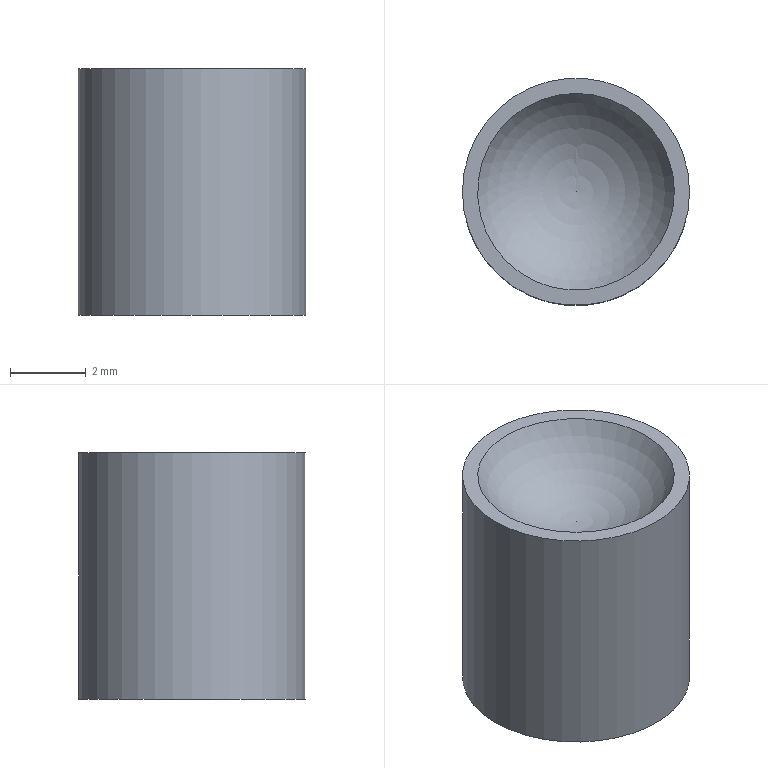Component | NX | DXF_02_SPRING_BRACKET | 1 solid | 4 faces | box 6 x 6 x 6.5 mm | volume 166 mm3 | plane 2 | cylinder 1 | sphere 1 | commonest cylinder face diameters 6 x1
STEP:
#1=CARTESIAN_POINT('',(0.,0.,0.));
#2=DIRECTION('',(0.,0.,1.));
#3=DIRECTION('',(1.,0.,0.));
#4=AXIS2_PLACEMENT_3D('',#1,#2,#3);
#5=CARTESIAN_POINT('',(3.,-0.,27.531));
#6=VERTEX_POINT('',#5);
#7=CARTESIAN_POINT('',(0.,-0.,27.531));
#8=DIRECTION('',(0.,0.,-1.));
#9=DIRECTION('',(1.,0.,0.));
#10=AXIS2_PLACEMENT_3D('',#7,#8,#9);
#11=CIRCLE('',#10,3.);
#12=CARTESIAN_POINT('',(0.,-0.,17.531));
#13=DIRECTION('',(0.,0.,1.));
#14=DIRECTION('',(1.,0.,0.));
#15=AXIS2_PLACEMENT_3D('',#12,#13,#14);
#16=CYLINDRICAL_SURFACE('',#15,3.);
#17=CARTESIAN_POINT('',(6.283,10.));
#18=DIRECTION('',(-1.,0.));
#19=VECTOR('',#18,1.);
#20=LINE('',#17,#19);
#21=(GEOMETRIC_REPRESENTATION_CONTEXT(2)PARAMETRIC_REPRESENTATION_CONTEXT()REPRESENTATION_CONTEXT('',''));
#22=DEFINITIONAL_REPRESENTATION('',(#20),#21);
#23=PCURVE('',#16,#22);
#24=CARTESIAN_POINT('',(0.,-0.,27.531));
#25=DIRECTION('',(0.,0.,1.));
#26=DIRECTION('',(1.,0.,0.));
#27=AXIS2_PLACEMENT_3D('',#24,#25,#26);
#28=PLANE('',#27);
#29=CARTESIAN_POINT('',(3.,0.));
#30=CARTESIAN_POINT('',(3.,-5.196));
#31=CARTESIAN_POINT('',(-1.5,-2.598));
#32=CARTESIAN_POINT('',(-6.,-0.));
#33=CARTESIAN_POINT('',(-1.5,2.598));
#34=CARTESIAN_POINT('',(3.,5.196));
#35=CARTESIAN_POINT('',(3.,0.));
#36=(BOUNDED_CURVE()B_SPLINE_CURVE(2,(#29,#30,#31,#32,#33,#34,#35),.UNSPECIFIED.,.T.,.F.)B_SPLINE_CURVE_WITH_KNOTS((1,2,2,2,2,1),(-2.094,0.,2.094,4.189,6.283,8.378),.UNSPECIFIED.)CURVE()GEOMETRIC_REPRESENTATION_ITEM()RATIONAL_B_SPLINE_CURVE((1.,0.5,1.,0.5,1.,0.5,1.))REPRESENTATION_ITEM(''));
#37=(GEOMETRIC_REPRESENTATION_CONTEXT(2)PARAMETRIC_REPRESENTATION_CONTEXT()REPRESENTATION_CONTEXT('',''));
#38=DEFINITIONAL_REPRESENTATION('',(#36),#37);
#39=PCURVE('',#28,#38);
#40=SURFACE_CURVE('',#11,(#23,#39),.PCURVE_S1.);
#41=EDGE_CURVE('',#6,#6,#40,.T.);
#42=ORIENTED_EDGE('',*,*,#41,.T.);
#43=CARTESIAN_POINT('',(3.,-0.,21.031));
#44=VERTEX_POINT('',#43);
#45=CARTESIAN_POINT('',(3.,-0.,21.031));
#46=CARTESIAN_POINT('',(3.,-0.,27.531));
#47=B_SPLINE_CURVE_WITH_KNOTS('',1,(#45,#46),.UNSPECIFIED.,.F.,.F.,(2,2),(3.5,10.),.PIECEWISE_BEZIER_KNOTS.);
#48=CARTESIAN_POINT('',(0.,0.));
#49=DIRECTION('',(0.,1.));
#50=VECTOR('',#49,1.);
#51=LINE('',#48,#50);
#52=(GEOMETRIC_REPRESENTATION_CONTEXT(2)PARAMETRIC_REPRESENTATION_CONTEXT()REPRESENTATION_CONTEXT('',''));
#53=DEFINITIONAL_REPRESENTATION('',(#51),#52);
#54=PCURVE('',#16,#53);
#55=CARTESIAN_POINT('',(6.283,0.));
#56=DIRECTION('',(0.,1.));
#57=VECTOR('',#56,1.);
#58=LINE('',#55,#57);
#59=(GEOMETRIC_REPRESENTATION_CONTEXT(2)PARAMETRIC_REPRESENTATION_CONTEXT()REPRESENTATION_CONTEXT('',''));
#60=DEFINITIONAL_REPRESENTATION('',(#58),#59);
#61=PCURVE('',#16,#60);
#62=SEAM_CURVE('',#47,(#54,#61),.PCURVE_S1.);
#63=EDGE_CURVE('',#44,#6,#62,.T.);
#64=ORIENTED_EDGE('',*,*,#63,.F.);
#65=CARTESIAN_POINT('',(-3.,-0.,21.031));
#66=VERTEX_POINT('',#65);
#67=CARTESIAN_POINT('',(0.,-0.,21.031));
#68=DIRECTION('',(0.,0.,1.));
#69=DIRECTION('',(-1.,0.,0.));
#70=AXIS2_PLACEMENT_3D('',#67,#68,#69);
#71=CIRCLE('',#70,3.);
#72=CARTESIAN_POINT('',(-3.142,3.5));
#73=DIRECTION('',(1.,0.));
#74=VECTOR('',#73,1.);
#75=LINE('',#72,#74);
#76=(GEOMETRIC_REPRESENTATION_CONTEXT(2)PARAMETRIC_REPRESENTATION_CONTEXT()REPRESENTATION_CONTEXT('',''));
#77=DEFINITIONAL_REPRESENTATION('',(#75),#76);
#78=PCURVE('',#16,#77);
#79=CARTESIAN_POINT('',(0.,-0.,21.031));
#80=DIRECTION('',(0.,0.,-1.));
#81=DIRECTION('',(-1.,0.,0.));
#82=AXIS2_PLACEMENT_3D('',#79,#80,#81);
#83=PLANE('',#82);
#84=CARTESIAN_POINT('',(3.,0.));
#85=CARTESIAN_POINT('',(3.,-5.196));
#86=CARTESIAN_POINT('',(-1.5,-2.598));
#87=CARTESIAN_POINT('',(-6.,-0.));
#88=CARTESIAN_POINT('',(-1.5,2.598));
#89=CARTESIAN_POINT('',(3.,5.196));
#90=CARTESIAN_POINT('',(3.,0.));
#91=(BOUNDED_CURVE()B_SPLINE_CURVE(2,(#84,#85,#86,#87,#88,#89,#90),.UNSPECIFIED.,.T.,.F.)B_SPLINE_CURVE_WITH_KNOTS((1,2,2,2,2,1),(-2.094,0.,2.094,4.189,6.283,8.378),.UNSPECIFIED.)CURVE()GEOMETRIC_REPRESENTATION_ITEM()RATIONAL_B_SPLINE_CURVE((1.,0.5,1.,0.5,1.,0.5,1.))REPRESENTATION_ITEM(''));
#92=(GEOMETRIC_REPRESENTATION_CONTEXT(2)PARAMETRIC_REPRESENTATION_CONTEXT()REPRESENTATION_CONTEXT('',''));
#93=DEFINITIONAL_REPRESENTATION('',(#91),#92);
#94=PCURVE('',#83,#93);
#95=SURFACE_CURVE('',#71,(#78,#94),.PCURVE_S1.);
#96=EDGE_CURVE('',#44,#66,#95,.T.);
#97=ORIENTED_EDGE('',*,*,#96,.T.);
#98=CARTESIAN_POINT('',(0.,-0.,21.031));
#99=DIRECTION('',(0.,0.,1.));
#100=DIRECTION('',(-1.,0.,0.));
#101=AXIS2_PLACEMENT_3D('',#98,#99,#100);
#102=CIRCLE('',#101,3.);
#103=CARTESIAN_POINT('',(3.142,3.5));
#104=DIRECTION('',(1.,0.));
#105=VECTOR('',#104,1.);
#106=LINE('',#103,#105);
#107=(GEOMETRIC_REPRESENTATION_CONTEXT(2)PARAMETRIC_REPRESENTATION_CONTEXT()REPRESENTATION_CONTEXT('',''));
#108=DEFINITIONAL_REPRESENTATION('',(#106),#107);
#109=PCURVE('',#16,#108);
#110=CARTESIAN_POINT('',(3.,0.));
#111=CARTESIAN_POINT('',(3.,-5.196));
#112=CARTESIAN_POINT('',(-1.5,-2.598));
#113=CARTESIAN_POINT('',(-6.,-0.));
#114=CARTESIAN_POINT('',(-1.5,2.598));
#115=CARTESIAN_POINT('',(3.,5.196));
#116=CARTESIAN_POINT('',(3.,0.));
#117=(BOUNDED_CURVE()B_SPLINE_CURVE(2,(#110,#111,#112,#113,#114,#115,#116),.UNSPECIFIED.,.T.,.F.)B_SPLINE_CURVE_WITH_KNOTS((1,2,2,2,2,1),(-2.094,0.,2.094,4.189,6.283,8.378),.UNSPECIFIED.)CURVE()GEOMETRIC_REPRESENTATION_ITEM()RATIONAL_B_SPLINE_CURVE((1.,0.5,1.,0.5,1.,0.5,1.))REPRESENTATION_ITEM(''));
#118=(GEOMETRIC_REPRESENTATION_CONTEXT(2)PARAMETRIC_REPRESENTATION_CONTEXT()REPRESENTATION_CONTEXT('',''));
#119=DEFINITIONAL_REPRESENTATION('',(#117),#118);
#120=PCURVE('',#83,#119);
#121=SURFACE_CURVE('',#102,(#109,#120),.PCURVE_S1.);
#122=EDGE_CURVE('',#66,#44,#121,.T.);
#123=ORIENTED_EDGE('',*,*,#122,.T.);
#124=ORIENTED_EDGE('',*,*,#63,.T.);
#125=EDGE_LOOP('',(#42,#64,#97,#123,#124));
#126=FACE_BOUND('',#125,.T.);
#127=ADVANCED_FACE('',(#126),#16,.T.);
#128=ORIENTED_EDGE('',*,*,#122,.F.);
#129=ORIENTED_EDGE('',*,*,#96,.F.);
#130=EDGE_LOOP('',(#128,#129));
#131=FACE_BOUND('',#130,.T.);
#132=ADVANCED_FACE('',(#131),#83,.T.);
#133=CARTESIAN_POINT('',(2.598,-0.,27.531));
#134=VERTEX_POINT('',#133);
#135=CARTESIAN_POINT('',(0.,2.598,27.531));
#136=VERTEX_POINT('',#135);
#137=CARTESIAN_POINT('',(0.,-0.,27.531));
#138=DIRECTION('',(0.,0.,-1.));
#139=DIRECTION('',(1.,0.,0.));
#140=AXIS2_PLACEMENT_3D('',#137,#138,#139);
#141=CIRCLE('',#140,2.598);
#142=CARTESIAN_POINT('',(2.598,0.));
#143=CARTESIAN_POINT('',(2.598,-4.5));
#144=CARTESIAN_POINT('',(-1.299,-2.25));
#145=CARTESIAN_POINT('',(-5.196,-0.));
#146=CARTESIAN_POINT('',(-1.299,2.25));
#147=CARTESIAN_POINT('',(2.598,4.5));
#148=CARTESIAN_POINT('',(2.598,0.));
#149=(BOUNDED_CURVE()B_SPLINE_CURVE(2,(#142,#143,#144,#145,#146,#147,#148),.UNSPECIFIED.,.T.,.F.)B_SPLINE_CURVE_WITH_KNOTS((1,2,2,2,2,1),(-2.094,0.,2.094,4.189,6.283,8.378),.UNSPECIFIED.)CURVE()GEOMETRIC_REPRESENTATION_ITEM()RATIONAL_B_SPLINE_CURVE((1.,0.5,1.,0.5,1.,0.5,1.))REPRESENTATION_ITEM(''));
#150=(GEOMETRIC_REPRESENTATION_CONTEXT(2)PARAMETRIC_REPRESENTATION_CONTEXT()REPRESENTATION_CONTEXT('',''));
#151=DEFINITIONAL_REPRESENTATION('',(#149),#150);
#152=PCURVE('',#28,#151);
#153=CARTESIAN_POINT('',(0.,-0.,29.031));
#154=DIRECTION('',(0.,-0.,-1.));
#155=DIRECTION('',(0.,1.,-0.));
#156=AXIS2_PLACEMENT_3D('',#153,#154,#155);
#157=SPHERICAL_SURFACE('',#156,3.);
#158=CARTESIAN_POINT('',(1.571,0.5236));
#159=CARTESIAN_POINT('',(1.666,0.5236));
#160=CARTESIAN_POINT('',(1.856,0.5236));
#161=CARTESIAN_POINT('',(2.142,0.5236));
#162=CARTESIAN_POINT('',(2.428,0.5236));
#163=CARTESIAN_POINT('',(2.713,0.5236));
#164=CARTESIAN_POINT('',(2.999,0.5236));
#165=CARTESIAN_POINT('',(3.284,0.5236));
#166=CARTESIAN_POINT('',(3.57,0.5236));
#167=CARTESIAN_POINT('',(3.856,0.5236));
#168=CARTESIAN_POINT('',(4.141,0.5236));
#169=CARTESIAN_POINT('',(4.427,0.5236));
#170=CARTESIAN_POINT('',(4.712,0.5236));
#171=CARTESIAN_POINT('',(4.998,0.5236));
#172=CARTESIAN_POINT('',(5.284,0.5236));
#173=CARTESIAN_POINT('',(5.569,0.5236));
#174=CARTESIAN_POINT('',(5.855,0.5236));
#175=CARTESIAN_POINT('',(6.14,0.5236));
#176=CARTESIAN_POINT('',(6.426,0.5236));
#177=CARTESIAN_POINT('',(6.712,0.5236));
#178=CARTESIAN_POINT('',(6.997,0.5236));
#179=CARTESIAN_POINT('',(7.283,0.5236));
#180=CARTESIAN_POINT('',(7.568,0.5236));
#181=CARTESIAN_POINT('',(7.759,0.5236));
#182=CARTESIAN_POINT('',(7.854,0.5236));
#183=B_SPLINE_CURVE_WITH_KNOTS('',3,(#158,#159,#160,#161,#162,#163,#164,#165,#166,#167,#168,#169,#170,#171,#172,#173,#174,#175,#176,#177,#178,#179,#180,#181,#182),.UNSPECIFIED.,.F.,.F.,(4,1,1,1,1,1,1,1,1,1,1,1,1,1,1,1,1,1,1,1,1,1,4),(0.,0.2856,0.5712,0.8568,1.142,1.428,1.714,1.999,2.285,2.57,2.856,3.142,3.427,3.713,3.998,4.284,4.57,4.855,5.141,5.426,5.712,5.998,6.283),.QUASI_UNIFORM_KNOTS.);
#184=(GEOMETRIC_REPRESENTATION_CONTEXT(2)PARAMETRIC_REPRESENTATION_CONTEXT()REPRESENTATION_CONTEXT('',''));
#185=DEFINITIONAL_REPRESENTATION('',(#183),#184);
#186=PCURVE('',#157,#185);
#187=SURFACE_CURVE('',#141,(#152,#186),.PCURVE_S1.);
#188=EDGE_CURVE('',#134,#136,#187,.T.);
#189=ORIENTED_EDGE('',*,*,#188,.T.);
#190=CARTESIAN_POINT('',(0.,-0.,27.531));
#191=DIRECTION('',(0.,0.,-1.));
#192=DIRECTION('',(1.,0.,0.));
#193=AXIS2_PLACEMENT_3D('',#190,#191,#192);
#194=CIRCLE('',#193,2.598);
#195=CARTESIAN_POINT('',(2.598,0.));
#196=CARTESIAN_POINT('',(2.598,-4.5));
#197=CARTESIAN_POINT('',(-1.299,-2.25));
#198=CARTESIAN_POINT('',(-5.196,-0.));
#199=CARTESIAN_POINT('',(-1.299,2.25));
#200=CARTESIAN_POINT('',(2.598,4.5));
#201=CARTESIAN_POINT('',(2.598,0.));
#202=(BOUNDED_CURVE()B_SPLINE_CURVE(2,(#195,#196,#197,#198,#199,#200,#201),.UNSPECIFIED.,.T.,.F.)B_SPLINE_CURVE_WITH_KNOTS((1,2,2,2,2,1),(-2.094,0.,2.094,4.189,6.283,8.378),.UNSPECIFIED.)CURVE()GEOMETRIC_REPRESENTATION_ITEM()RATIONAL_B_SPLINE_CURVE((1.,0.5,1.,0.5,1.,0.5,1.))REPRESENTATION_ITEM(''));
#203=(GEOMETRIC_REPRESENTATION_CONTEXT(2)PARAMETRIC_REPRESENTATION_CONTEXT()REPRESENTATION_CONTEXT('',''));
#204=DEFINITIONAL_REPRESENTATION('',(#202),#203);
#205=PCURVE('',#28,#204);
#206=CARTESIAN_POINT('',(-4.712,0.5236));
#207=CARTESIAN_POINT('',(-4.617,0.5236));
#208=CARTESIAN_POINT('',(-4.427,0.5236));
#209=CARTESIAN_POINT('',(-4.141,0.5236));
#210=CARTESIAN_POINT('',(-3.856,0.5236));
#211=CARTESIAN_POINT('',(-3.57,0.5236));
#212=CARTESIAN_POINT('',(-3.284,0.5236));
#213=CARTESIAN_POINT('',(-2.999,0.5236));
#214=CARTESIAN_POINT('',(-2.713,0.5236));
#215=CARTESIAN_POINT('',(-2.428,0.5236));
#216=CARTESIAN_POINT('',(-2.142,0.5236));
#217=CARTESIAN_POINT('',(-1.856,0.5236));
#218=CARTESIAN_POINT('',(-1.571,0.5236));
#219=CARTESIAN_POINT('',(-1.285,0.5236));
#220=CARTESIAN_POINT('',(-0.9996,0.5236));
#221=CARTESIAN_POINT('',(-0.714,0.5236));
#222=CARTESIAN_POINT('',(-0.4284,0.5236));
#223=CARTESIAN_POINT('',(-0.1428,0.5236));
#224=CARTESIAN_POINT('',(0.1428,0.5236));
#225=CARTESIAN_POINT('',(0.4284,0.5236));
#226=CARTESIAN_POINT('',(0.714,0.5236));
#227=CARTESIAN_POINT('',(0.9996,0.5236));
#228=CARTESIAN_POINT('',(1.285,0.5236));
#229=CARTESIAN_POINT('',(1.476,0.5236));
#230=CARTESIAN_POINT('',(1.571,0.5236));
#231=B_SPLINE_CURVE_WITH_KNOTS('',3,(#206,#207,#208,#209,#210,#211,#212,#213,#214,#215,#216,#217,#218,#219,#220,#221,#222,#223,#224,#225,#226,#227,#228,#229,#230),.UNSPECIFIED.,.F.,.F.,(4,1,1,1,1,1,1,1,1,1,1,1,1,1,1,1,1,1,1,1,1,1,4),(0.,0.2856,0.5712,0.8568,1.142,1.428,1.714,1.999,2.285,2.57,2.856,3.142,3.427,3.713,3.998,4.284,4.57,4.855,5.141,5.426,5.712,5.998,6.283),.QUASI_UNIFORM_KNOTS.);
#232=(GEOMETRIC_REPRESENTATION_CONTEXT(2)PARAMETRIC_REPRESENTATION_CONTEXT()REPRESENTATION_CONTEXT('',''));
#233=DEFINITIONAL_REPRESENTATION('',(#231),#232);
#234=PCURVE('',#157,#233);
#235=SURFACE_CURVE('',#194,(#205,#234),.PCURVE_S1.);
#236=EDGE_CURVE('',#136,#134,#235,.T.);
#237=ORIENTED_EDGE('',*,*,#236,.T.);
#238=EDGE_LOOP('',(#189,#237));
#239=FACE_BOUND('',#238,.T.);
#240=ORIENTED_EDGE('',*,*,#41,.F.);
#241=EDGE_LOOP('',(#240));
#242=FACE_BOUND('',#241,.T.);
#243=ADVANCED_FACE('',(#239,#242),#28,.T.);
#244=ORIENTED_EDGE('',*,*,#188,.T.);
#245=CARTESIAN_POINT('',(0.,-0.,26.031));
#246=VERTEX_POINT('',#245);
#247=CARTESIAN_POINT('',(0.,2.598,27.531));
#248=CARTESIAN_POINT('',(0.,2.284,26.987));
#249=CARTESIAN_POINT('',(0.,1.827,26.525));
#250=CARTESIAN_POINT('',(0.,1.257,26.195));
#251=CARTESIAN_POINT('',(0.,0.6283,26.031));
#252=CARTESIAN_POINT('',(0.,-0.,26.031));
#253=B_SPLINE_CURVE_WITH_KNOTS('',5,(#247,#248,#249,#250,#251,#252),.UNSPECIFIED.,.F.,.F.,(6,6),(0.5236,1.571),.PIECEWISE_BEZIER_KNOTS.);
#254=CARTESIAN_POINT('',(6.283,0.));
#255=DIRECTION('',(0.,1.));
#256=VECTOR('',#255,1.);
#257=LINE('',#254,#256);
#258=(GEOMETRIC_REPRESENTATION_CONTEXT(2)PARAMETRIC_REPRESENTATION_CONTEXT()REPRESENTATION_CONTEXT('',''));
#259=DEFINITIONAL_REPRESENTATION('',(#257),#258);
#260=PCURVE('',#157,#259);
#261=CARTESIAN_POINT('',(0.,0.));
#262=DIRECTION('',(0.,1.));
#263=VECTOR('',#262,1.);
#264=LINE('',#261,#263);
#265=(GEOMETRIC_REPRESENTATION_CONTEXT(2)PARAMETRIC_REPRESENTATION_CONTEXT()REPRESENTATION_CONTEXT('',''));
#266=DEFINITIONAL_REPRESENTATION('',(#264),#265);
#267=PCURVE('',#157,#266);
#268=SEAM_CURVE('',#253,(#260,#267),.PCURVE_S1.);
#269=EDGE_CURVE('',#136,#246,#268,.T.);
#270=ORIENTED_EDGE('',*,*,#269,.T.);
#271=ORIENTED_EDGE('',*,*,#269,.F.);
#272=ORIENTED_EDGE('',*,*,#236,.T.);
#273=EDGE_LOOP('',(#244,#270,#271,#272));
#274=FACE_BOUND('',#273,.F.);
#275=ADVANCED_FACE('',(#274),#157,.F.);
#276=CLOSED_SHELL('',(#127,#132,#243,#275));
#277=MANIFOLD_SOLID_BREP('',#276);
#278=(LENGTH_UNIT()NAMED_UNIT(*)SI_UNIT(.MILLI.,.METRE.));
#279=UNCERTAINTY_MEASURE_WITH_UNIT(LENGTH_MEASURE(0.000005),#278,'','');
#280=(NAMED_UNIT(*)PLANE_ANGLE_UNIT()SI_UNIT($,.RADIAN.));
#281=(NAMED_UNIT(*)SI_UNIT($,.STERADIAN.)SOLID_ANGLE_UNIT());
#282=(GEOMETRIC_REPRESENTATION_CONTEXT(3)GLOBAL_UNCERTAINTY_ASSIGNED_CONTEXT((#279))GLOBAL_UNIT_ASSIGNED_CONTEXT((#278,#280,#281))REPRESENTATION_CONTEXT('',''));
#283=ADVANCED_BREP_SHAPE_REPRESENTATION('',(#4,#277),#282);